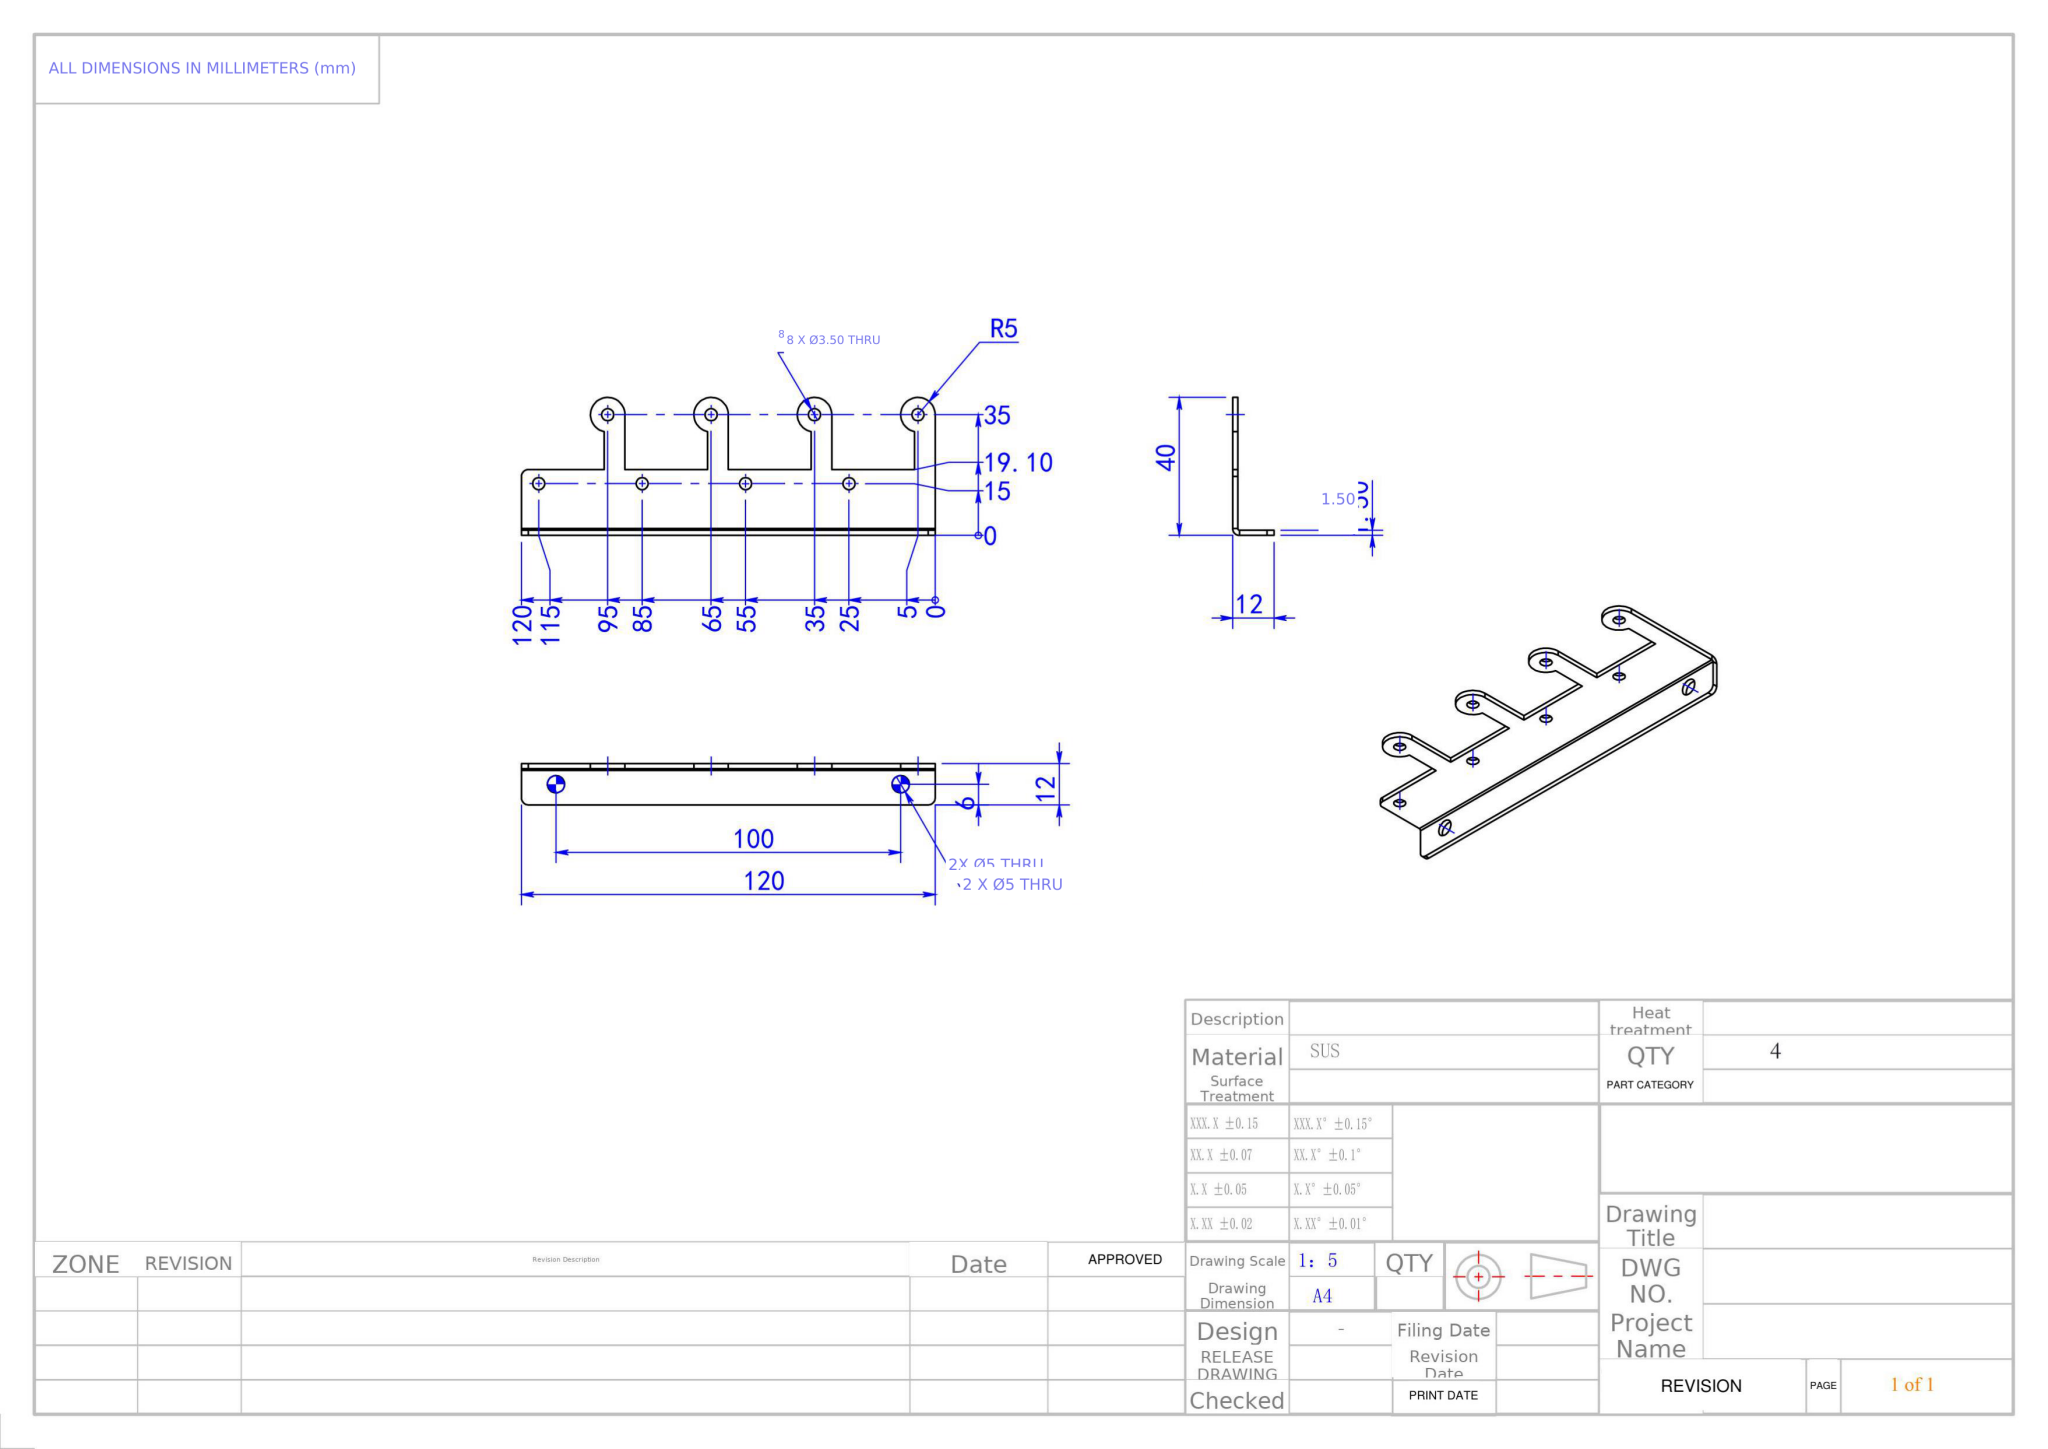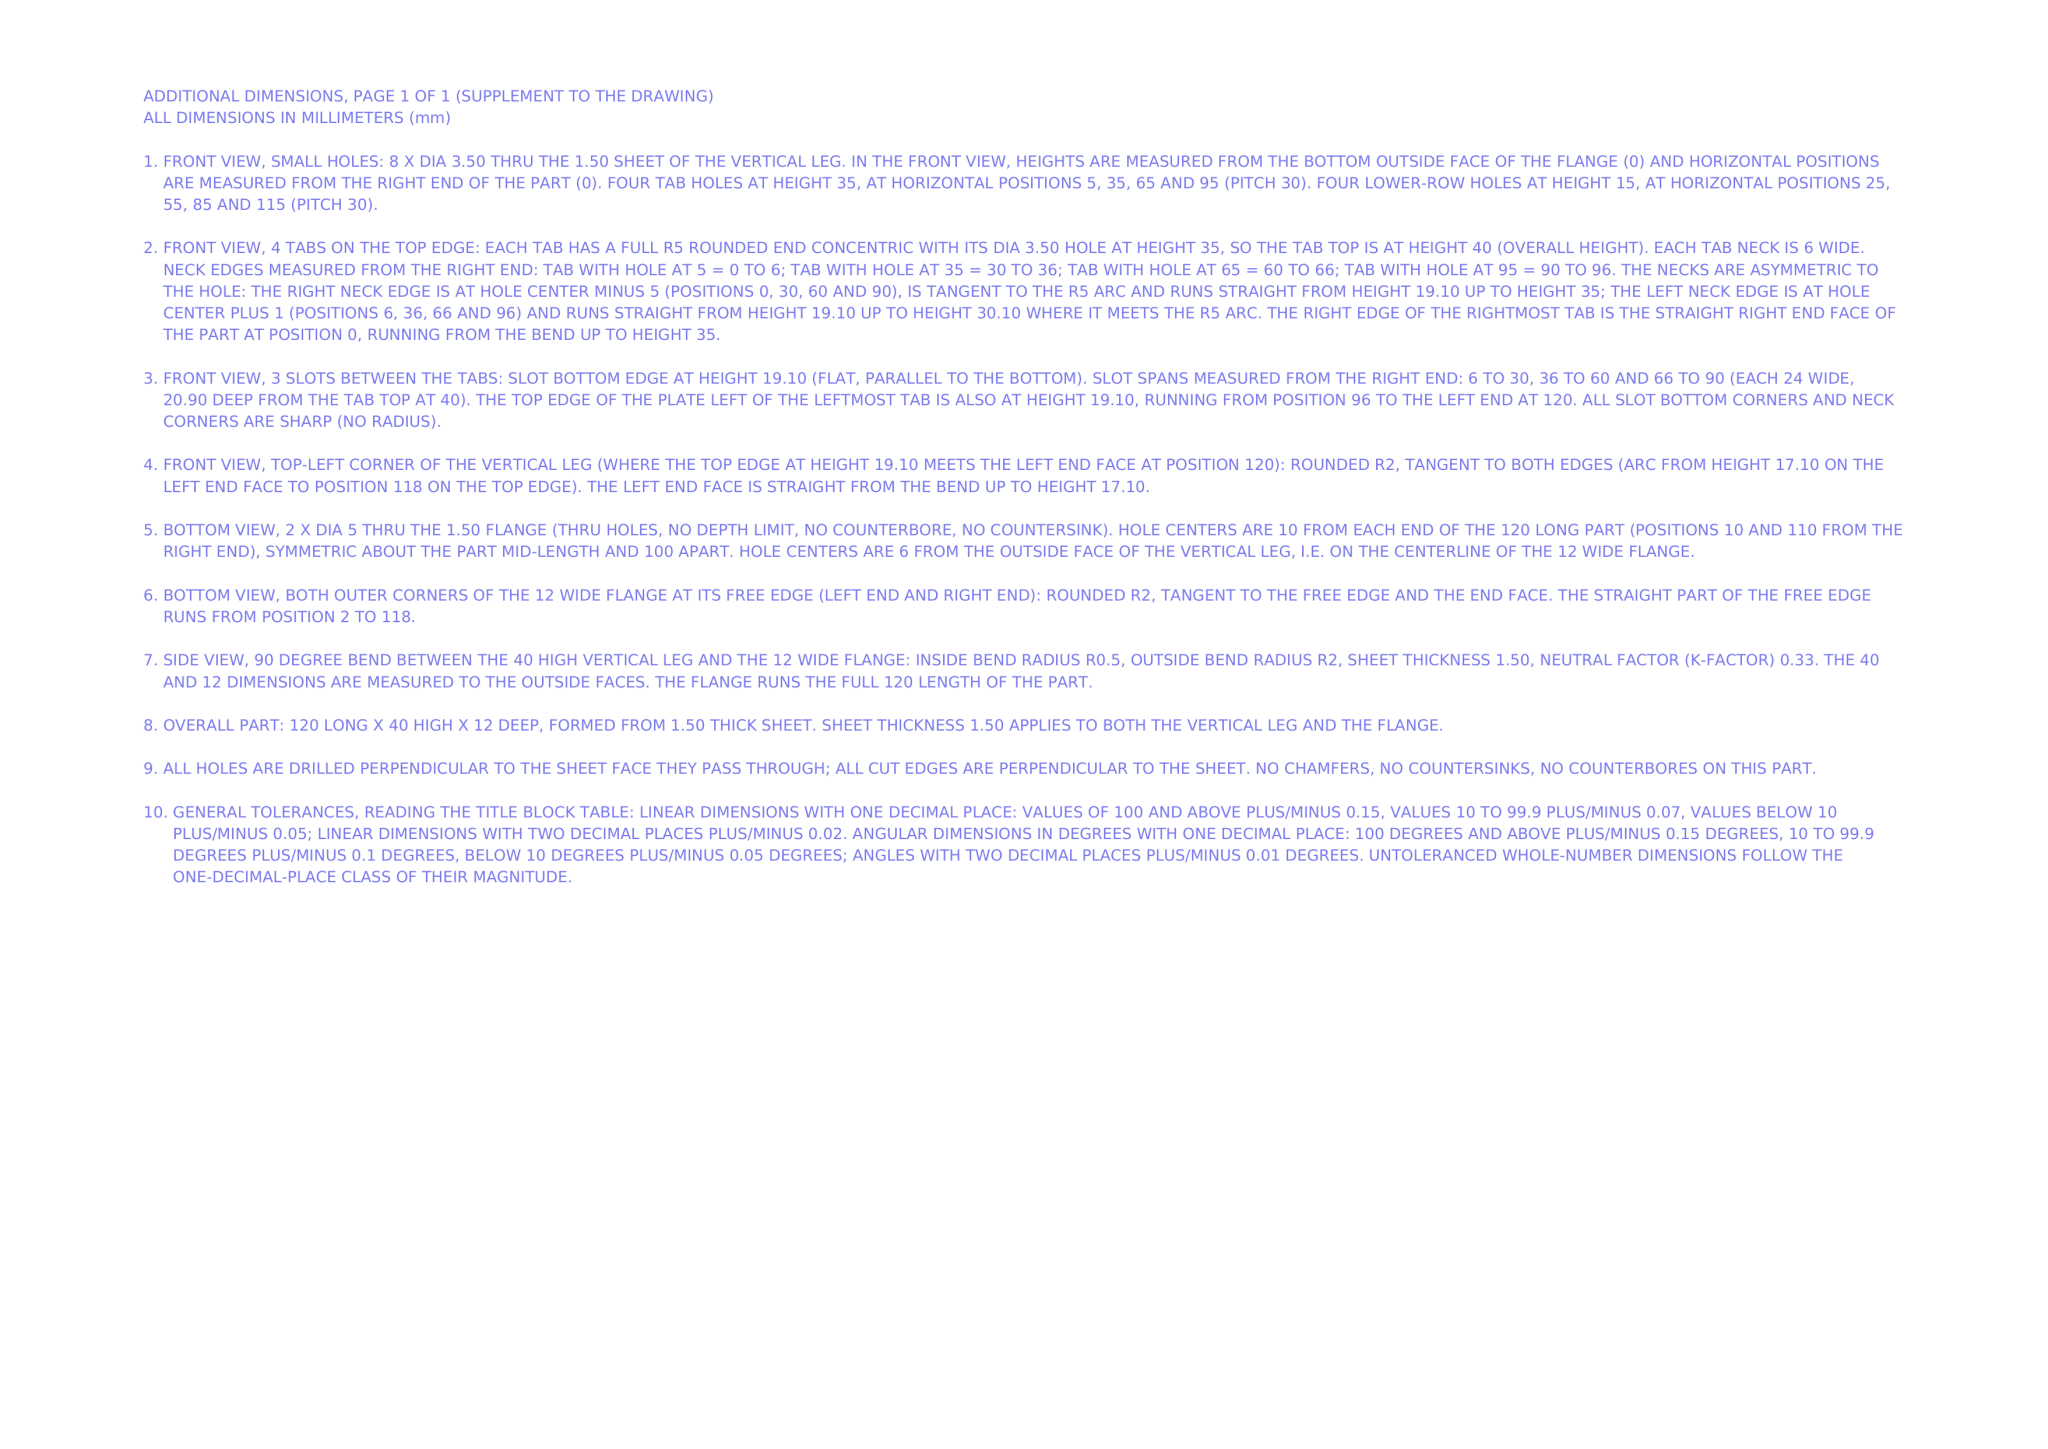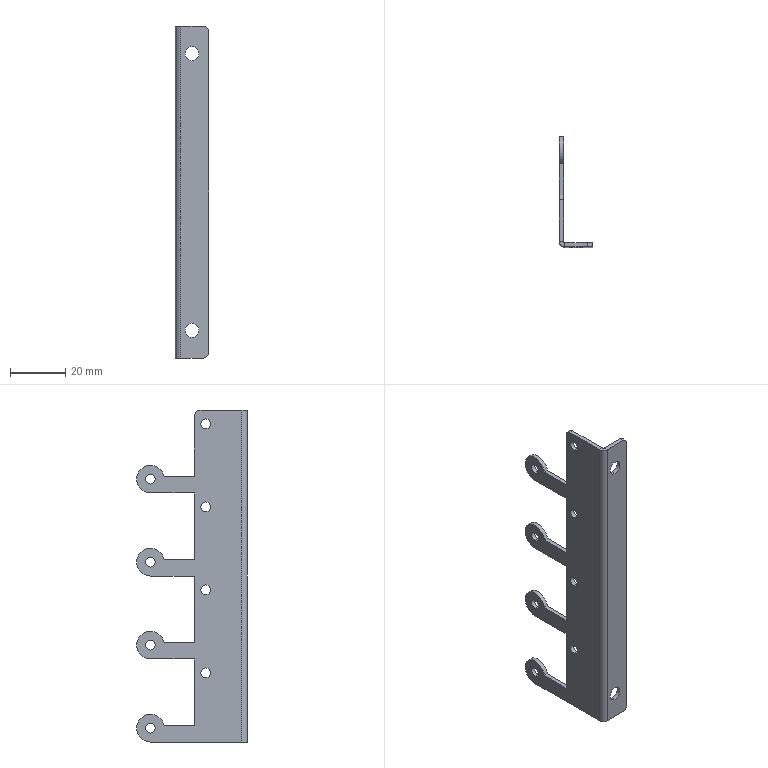Part | NX | mm | 1 solid | 51 faces | box 12 x 40 x 120 mm | volume 5949 mm3 | cylinder 29 | plane 22 | commonest cylinder face diameters 3.5 x16 5 x4 4 x4 10 x4 1 x1